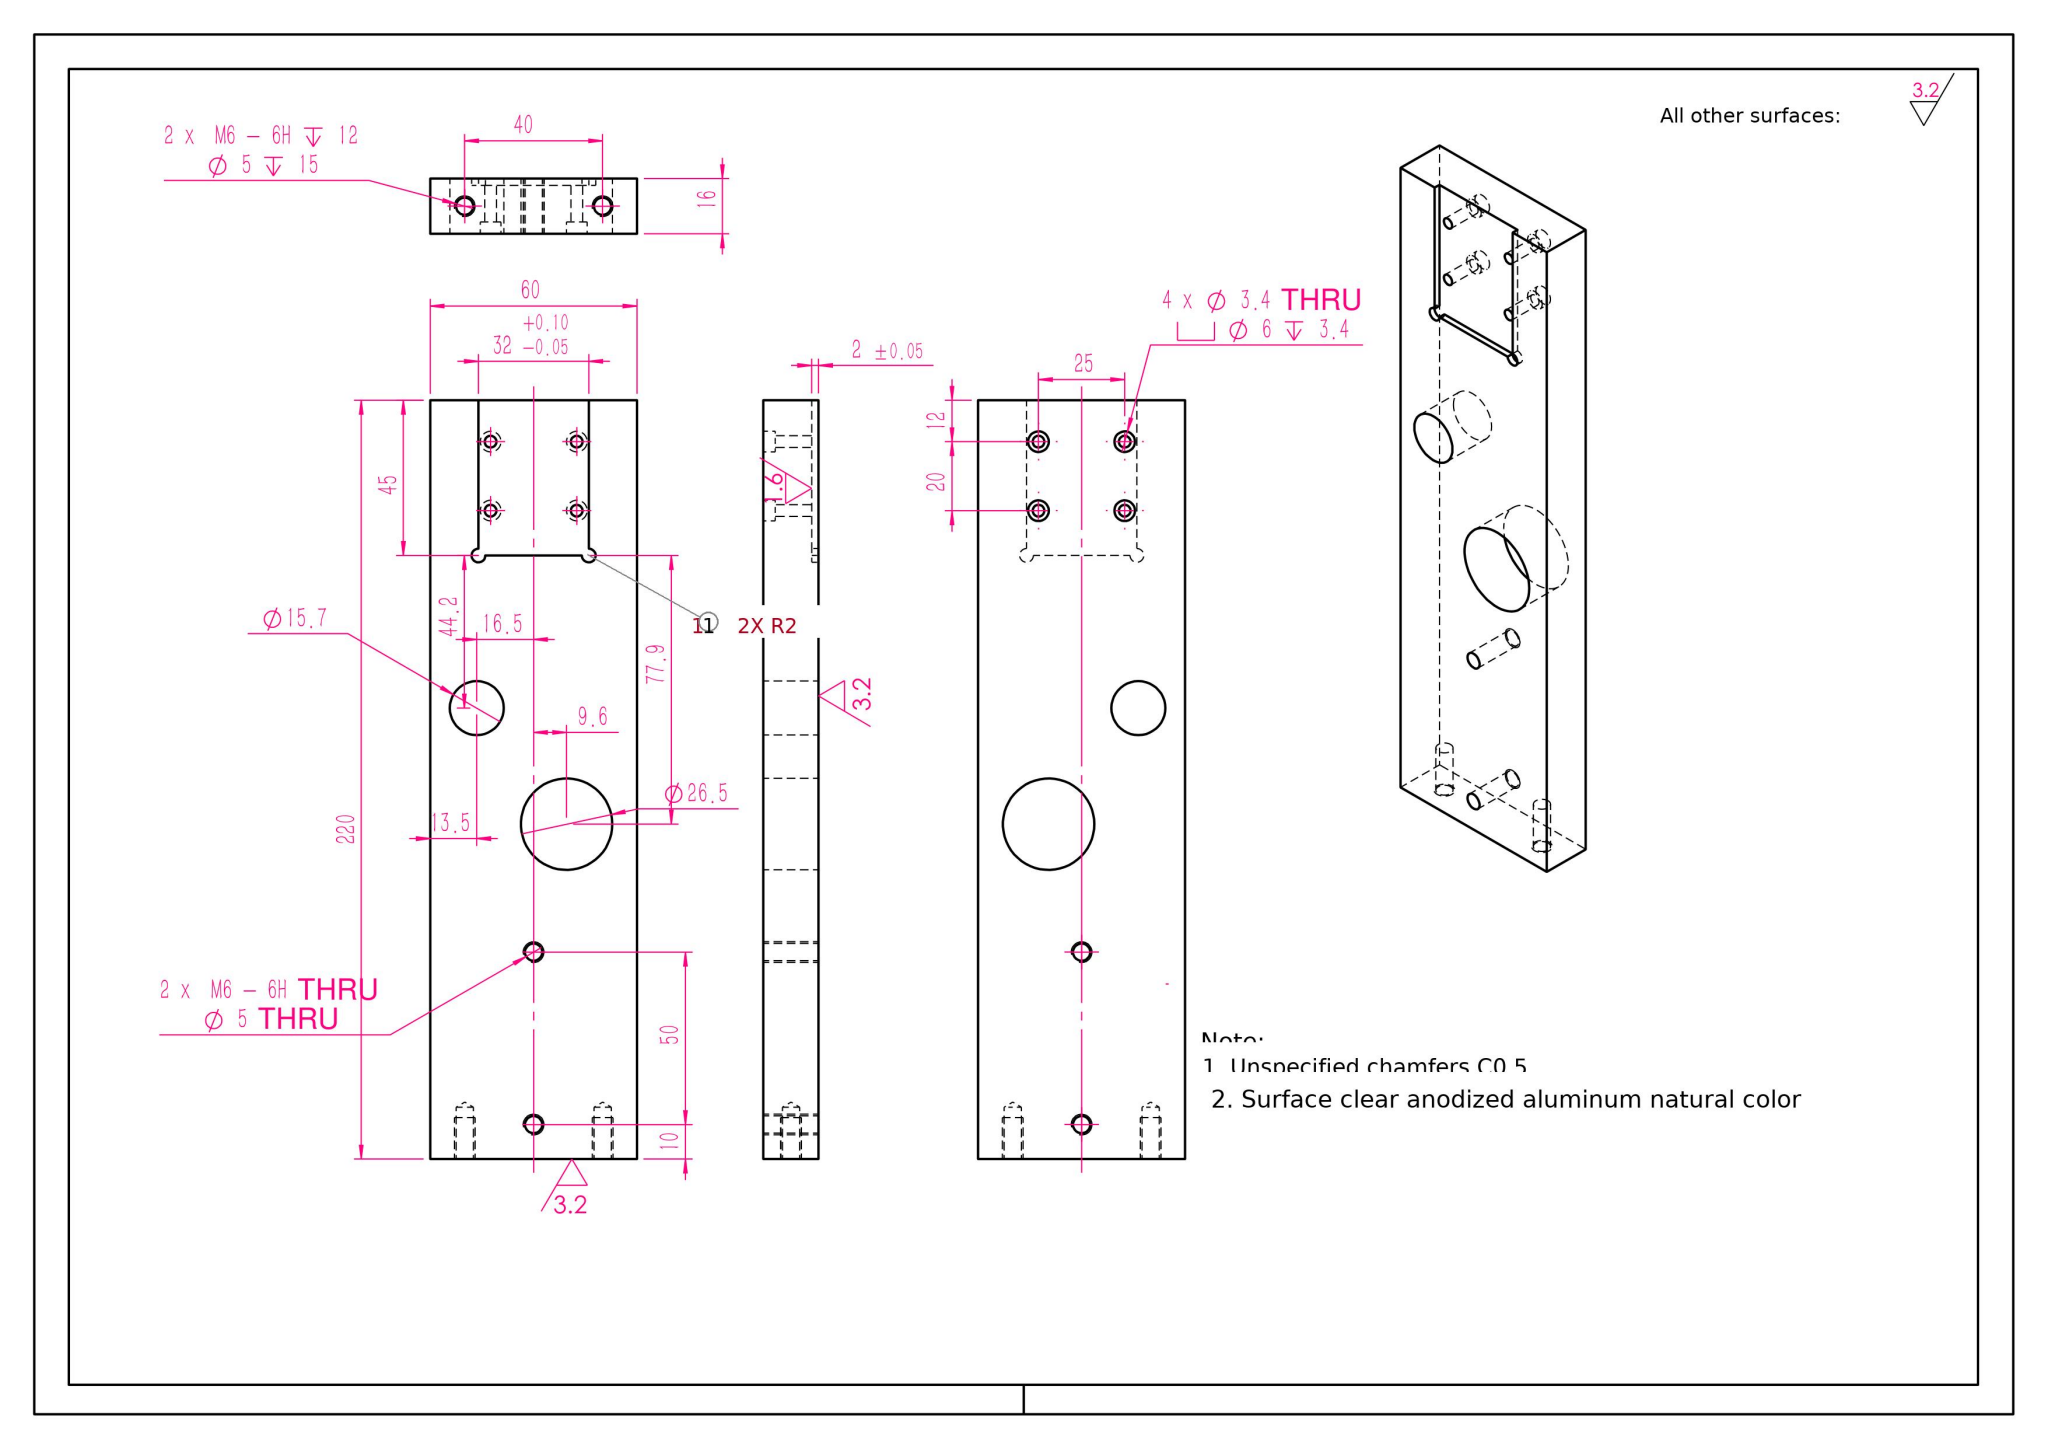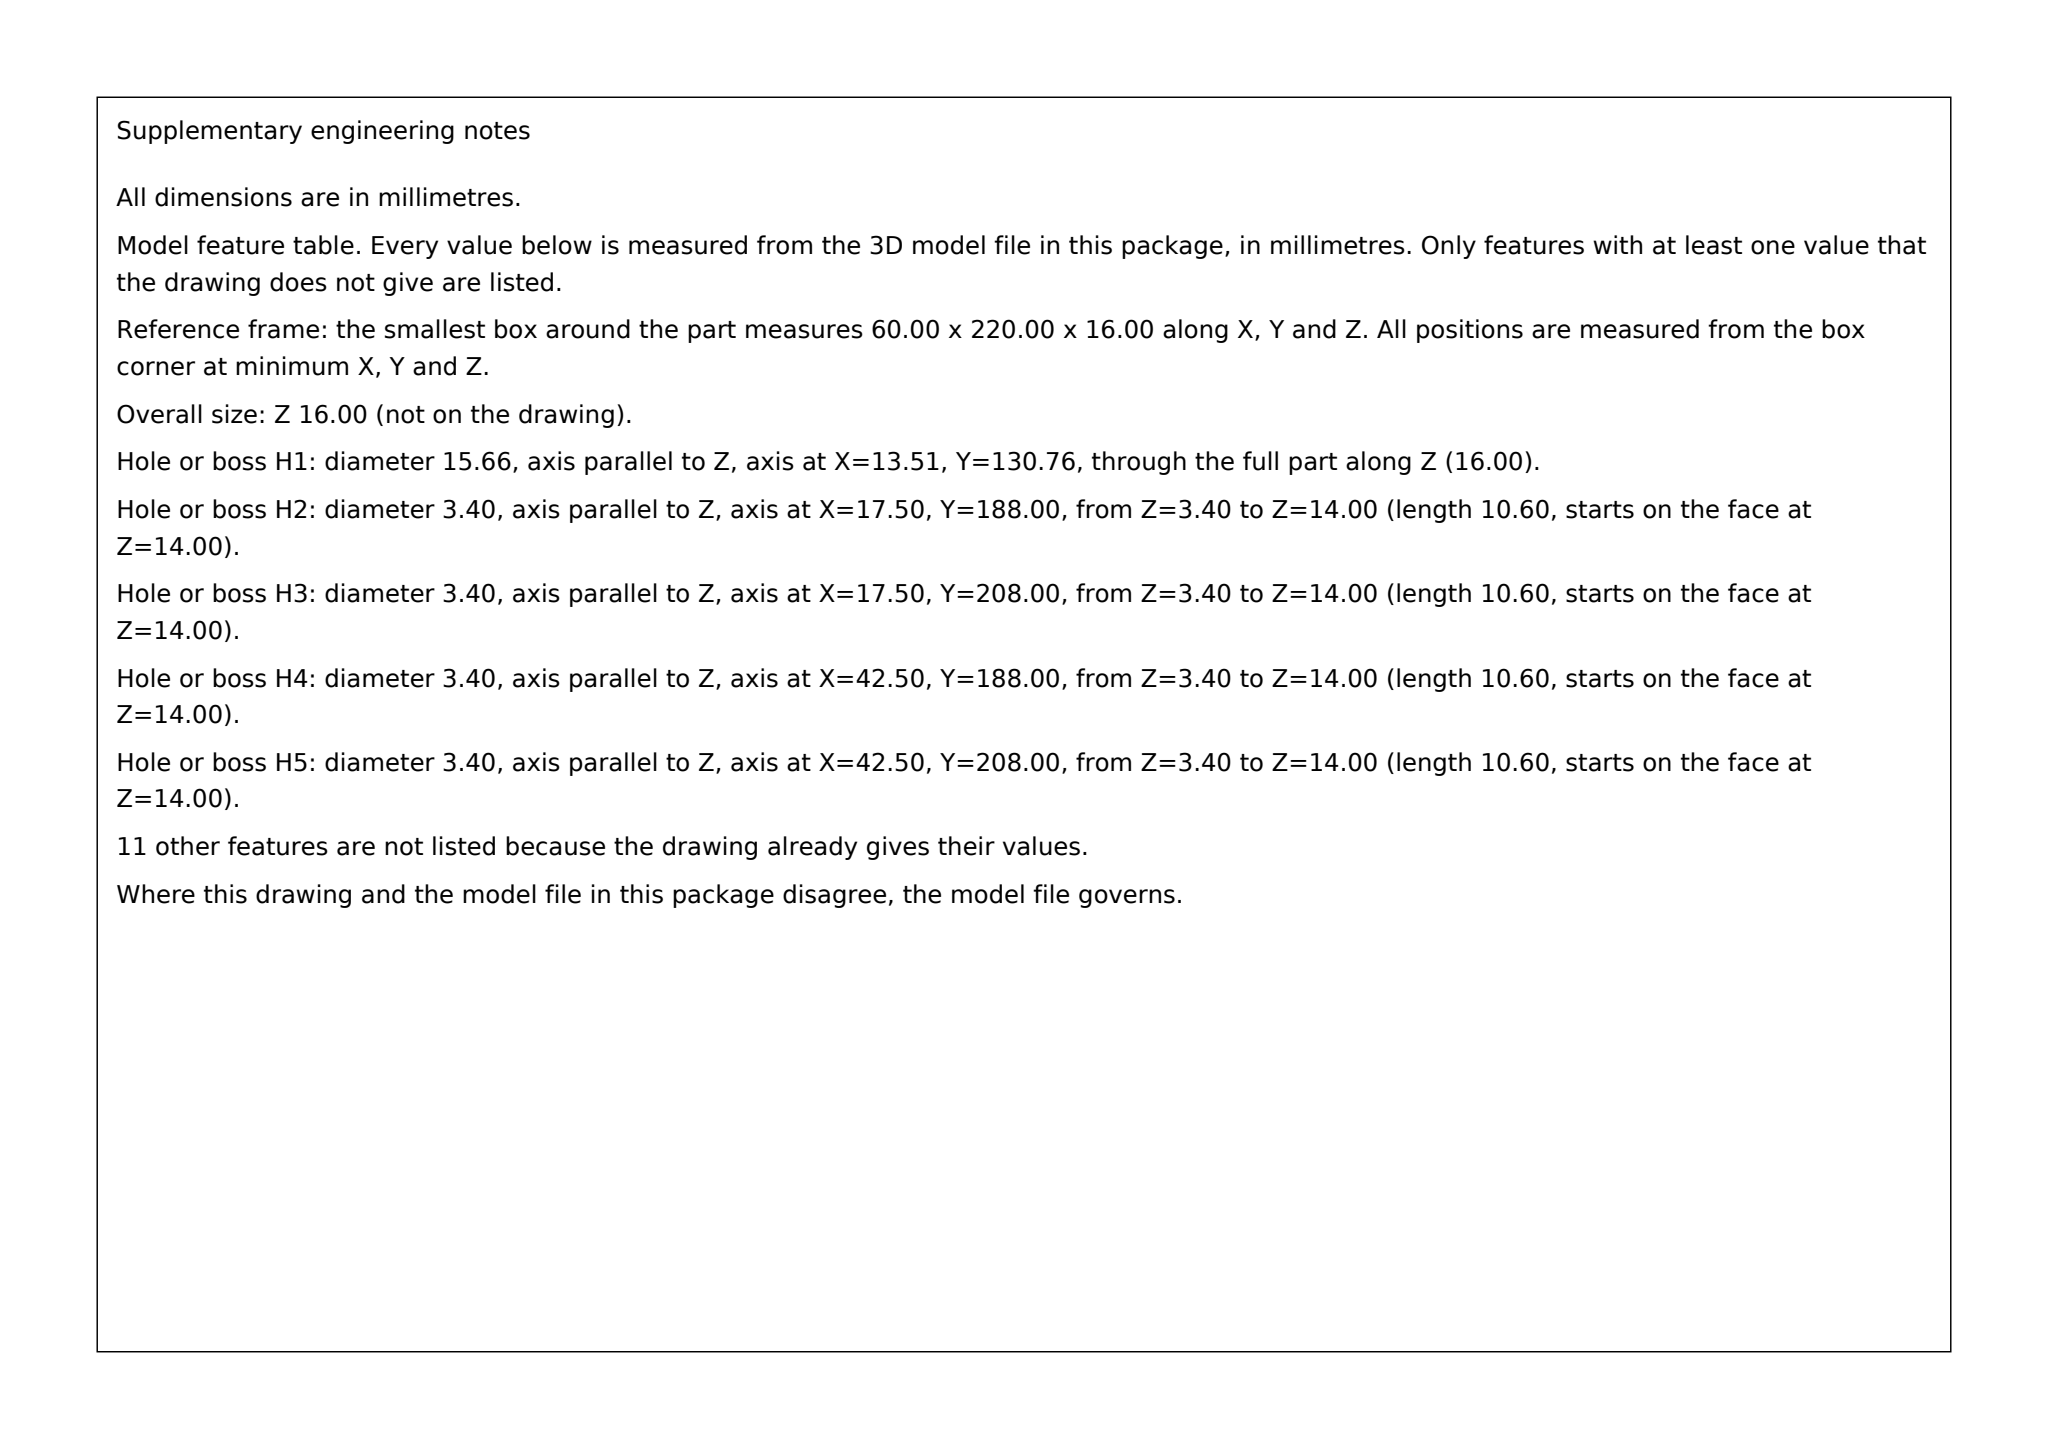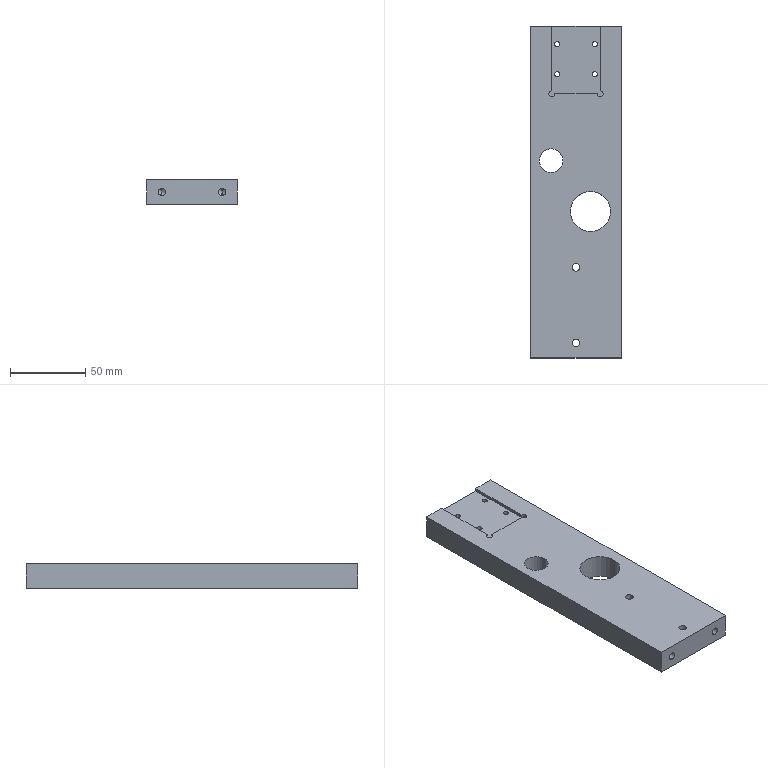Part | SolidWorks | mm | 1 solid | 49 faces | box 60 x 220 x 16 mm | volume 194353 mm3 | cylinder 31 | plane 14 | cone 4 | commonest cylinder face diameters 5 x8 6 x8 3.4 x8 4 x3 26.531 x2 15.65 x2
build123d program:
from build123d import *

# Parameters (mm, degrees)
SKETCH1_W                                            = 60
SKETCH1_H                                            = 220
BOSS_EXTRUDE1_DEPTH                                  = 16
M6_TAPPED_HOLE1_D                                    = 5
M6_TAPPED_HOLE1_DEPTH                                = 15
M6_TAPPED_HOLE1_TIP                                  = 1.502
SKETCH4_W                                            = 32
SKETCH4_H                                            = 90
CUT_EXTRUDE1_DEPTH                                   = 2
SKETCH5_R                                            = 2
CUT_EXTRUDE2_DEPTH                                   = 2
HOLE_SIZE_ACCORDING_TO_HEXAGON_SOCKET_HE_D           = 3.4
HOLE_SIZE_ACCORDING_TO_HEXAGON_SOCKET_HE_CBORE_D     = 6
HOLE_SIZE_ACCORDING_TO_HEXAGON_SOCKET_HE_CBORE_DEPTH = 3.4
M6_TAPPED_HOLE2_D                                    = 5
SKETCH10_R                                           = 13.265
SKETCH10_R_2                                         = 7.825
CUT_EXTRUDE3_DEPTH                                   = 80


with BuildPart() as part:
    # Sketch1 → Boss-Extrude1 (new body)
    with BuildSketch(Plane.XY):
        Rectangle(SKETCH1_W, SKETCH1_H)
    extrude(amount=BOSS_EXTRUDE1_DEPTH)

    # M6 Tapped Hole1
    with Locations(Plane(origin=(0, -110, 0), x_dir=(-1, 0, 0), z_dir=(0, -1, 0))):
        with Locations((20, -8), (-20, -8)):
            Hole(M6_TAPPED_HOLE1_D / 2, depth=M6_TAPPED_HOLE1_DEPTH)
            with Locations((0, 0, -(M6_TAPPED_HOLE1_DEPTH + M6_TAPPED_HOLE1_TIP / 2))):  # 118° drill point
                Cone(0, M6_TAPPED_HOLE1_D / 2, M6_TAPPED_HOLE1_TIP, mode=Mode.SUBTRACT)

    # Sketch4 → Cut-Extrude1 (cut)
    with BuildSketch(Plane.XY.offset(16)):
        with Locations((0, 110)):
            Rectangle(SKETCH4_W, SKETCH4_H)
    extrude(amount=-CUT_EXTRUDE1_DEPTH, mode=Mode.SUBTRACT)

    # Sketch5 → Cut-Extrude2 (cut)
    with BuildSketch(Plane.XY.offset(16)):
        with Locations((-16, 65)):
            Circle(SKETCH5_R)
        with Locations((16, 65)):
            Circle(SKETCH5_R)
    extrude(amount=-CUT_EXTRUDE2_DEPTH, mode=Mode.SUBTRACT)

    # Hole Size according to Hexagon Socket He (through all)
    with Locations(Plane(origin=(0, 0, 0), x_dir=(-1, 0, 0), z_dir=(0, 0, -1))):
        with Locations((-12.5, 98), (12.5, 98), (-12.5, 78), (12.5, 78)):
            CounterBoreHole(HOLE_SIZE_ACCORDING_TO_HEXAGON_SOCKET_HE_D / 2, HOLE_SIZE_ACCORDING_TO_HEXAGON_SOCKET_HE_CBORE_D / 2, HOLE_SIZE_ACCORDING_TO_HEXAGON_SOCKET_HE_CBORE_DEPTH)

    # M6 Tapped Hole2 (through all)
    with Locations(Plane(origin=(0, 0, 0), x_dir=(-1, 0, 0), z_dir=(0, 0, -1))):
        with Locations((0, -50), (0, -100)):
            Hole(M6_TAPPED_HOLE2_D / 2)

    # Sketch10 → Cut-Extrude3 (cut)
    with BuildSketch(Plane.XY.offset(16)):
        with Locations((9.57, -12.891)):
            Circle(SKETCH10_R)
        with Locations((-16.486, 20.759)):
            Circle(SKETCH10_R_2)
    extrude(amount=-CUT_EXTRUDE3_DEPTH, mode=Mode.SUBTRACT)


solid = part.part